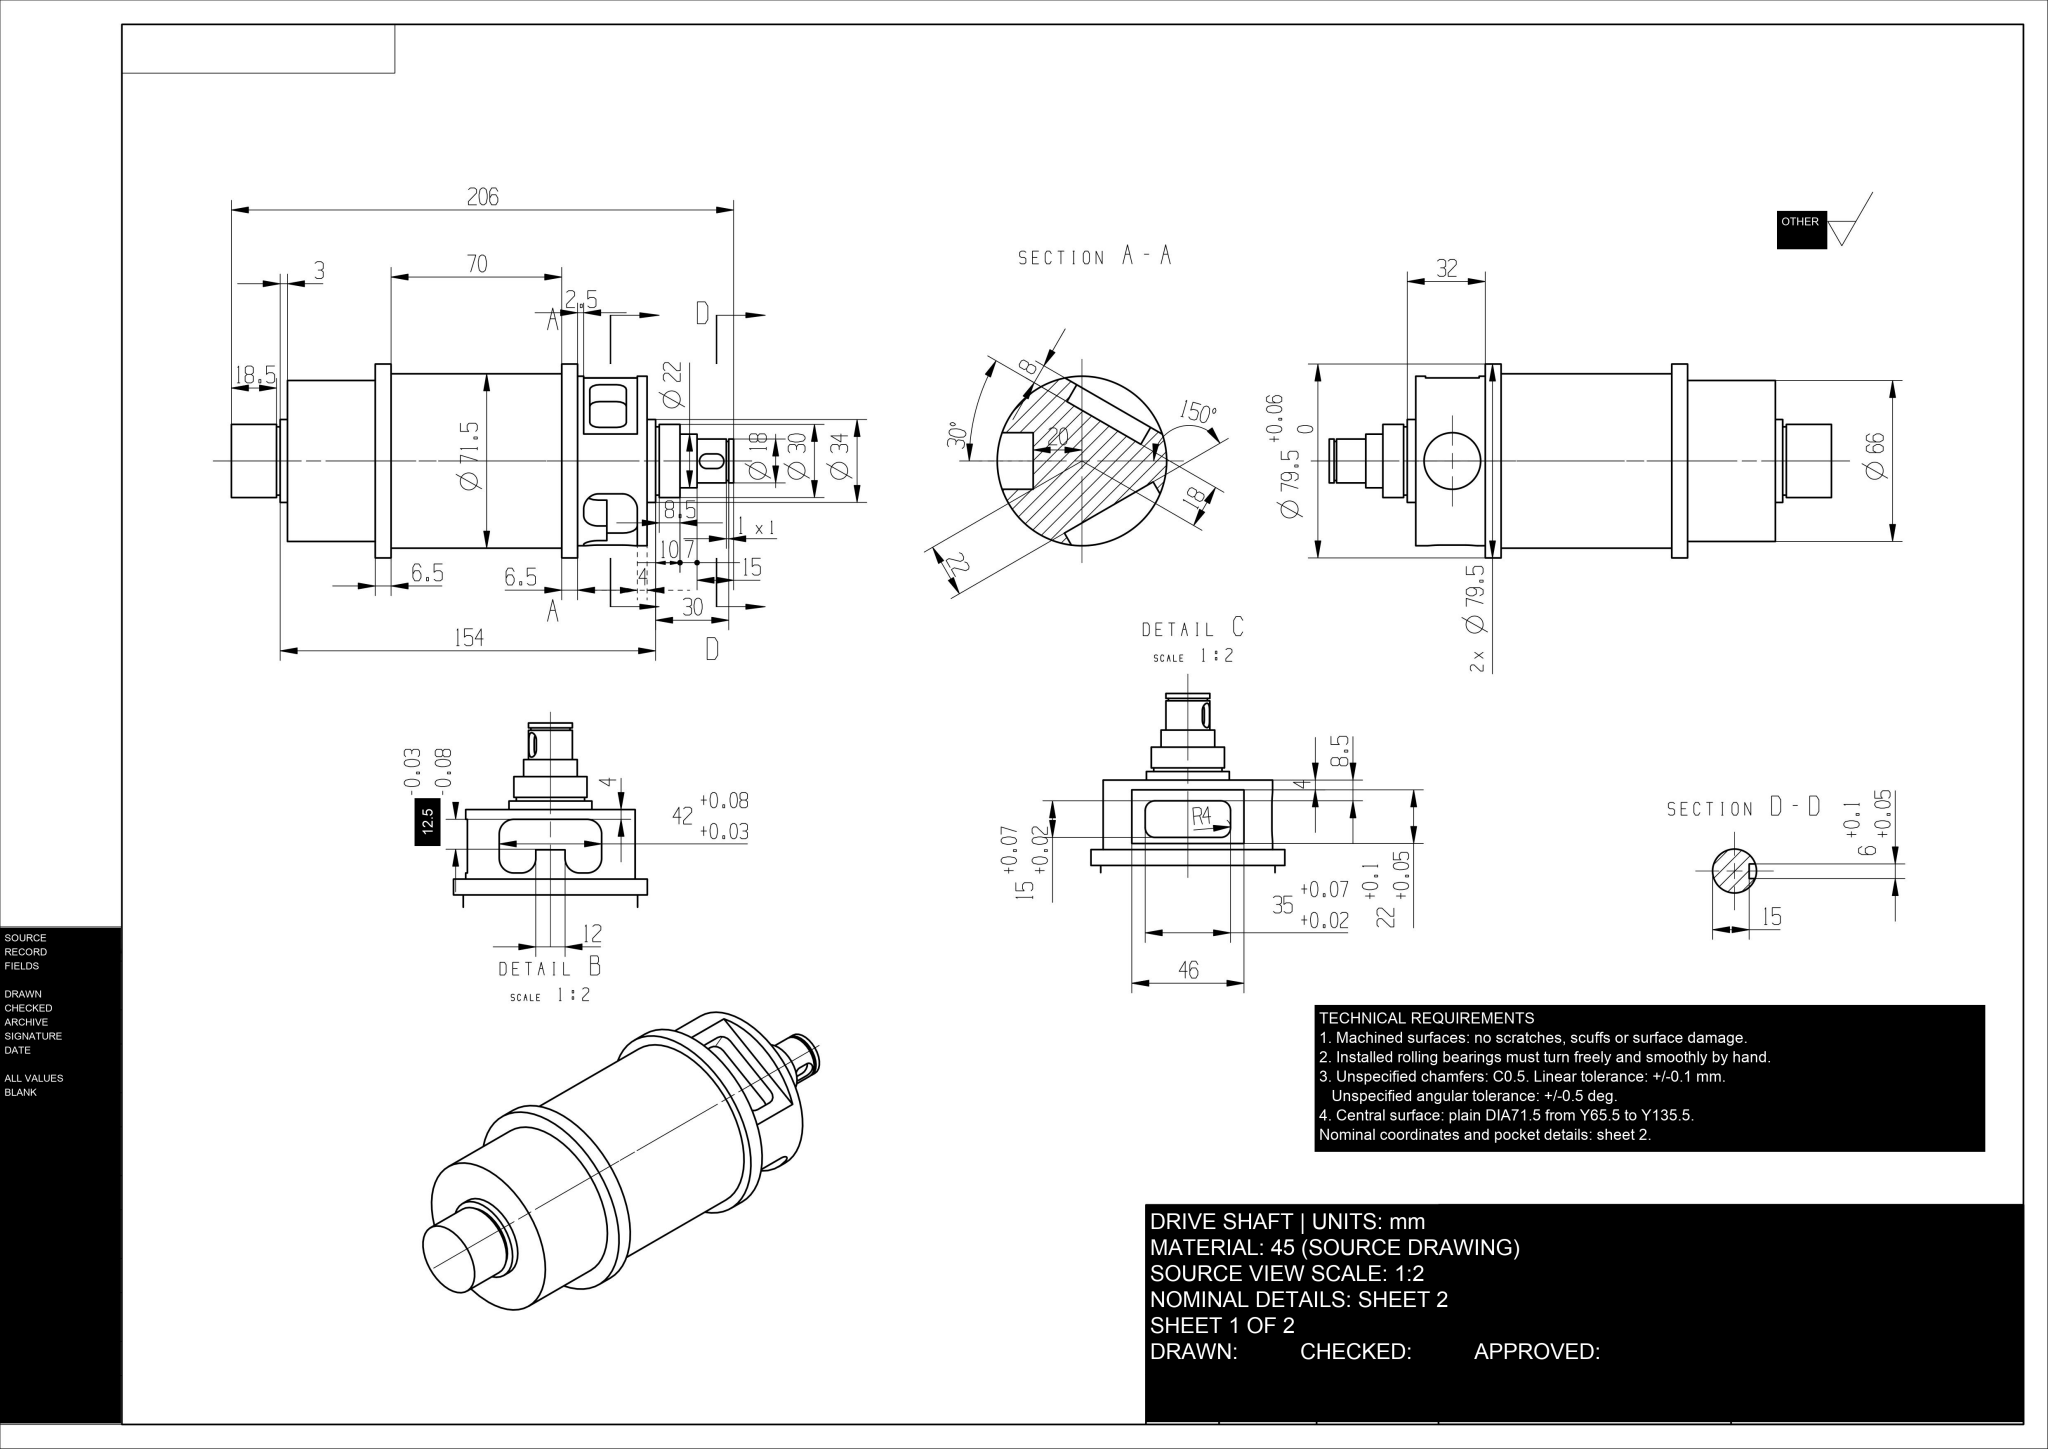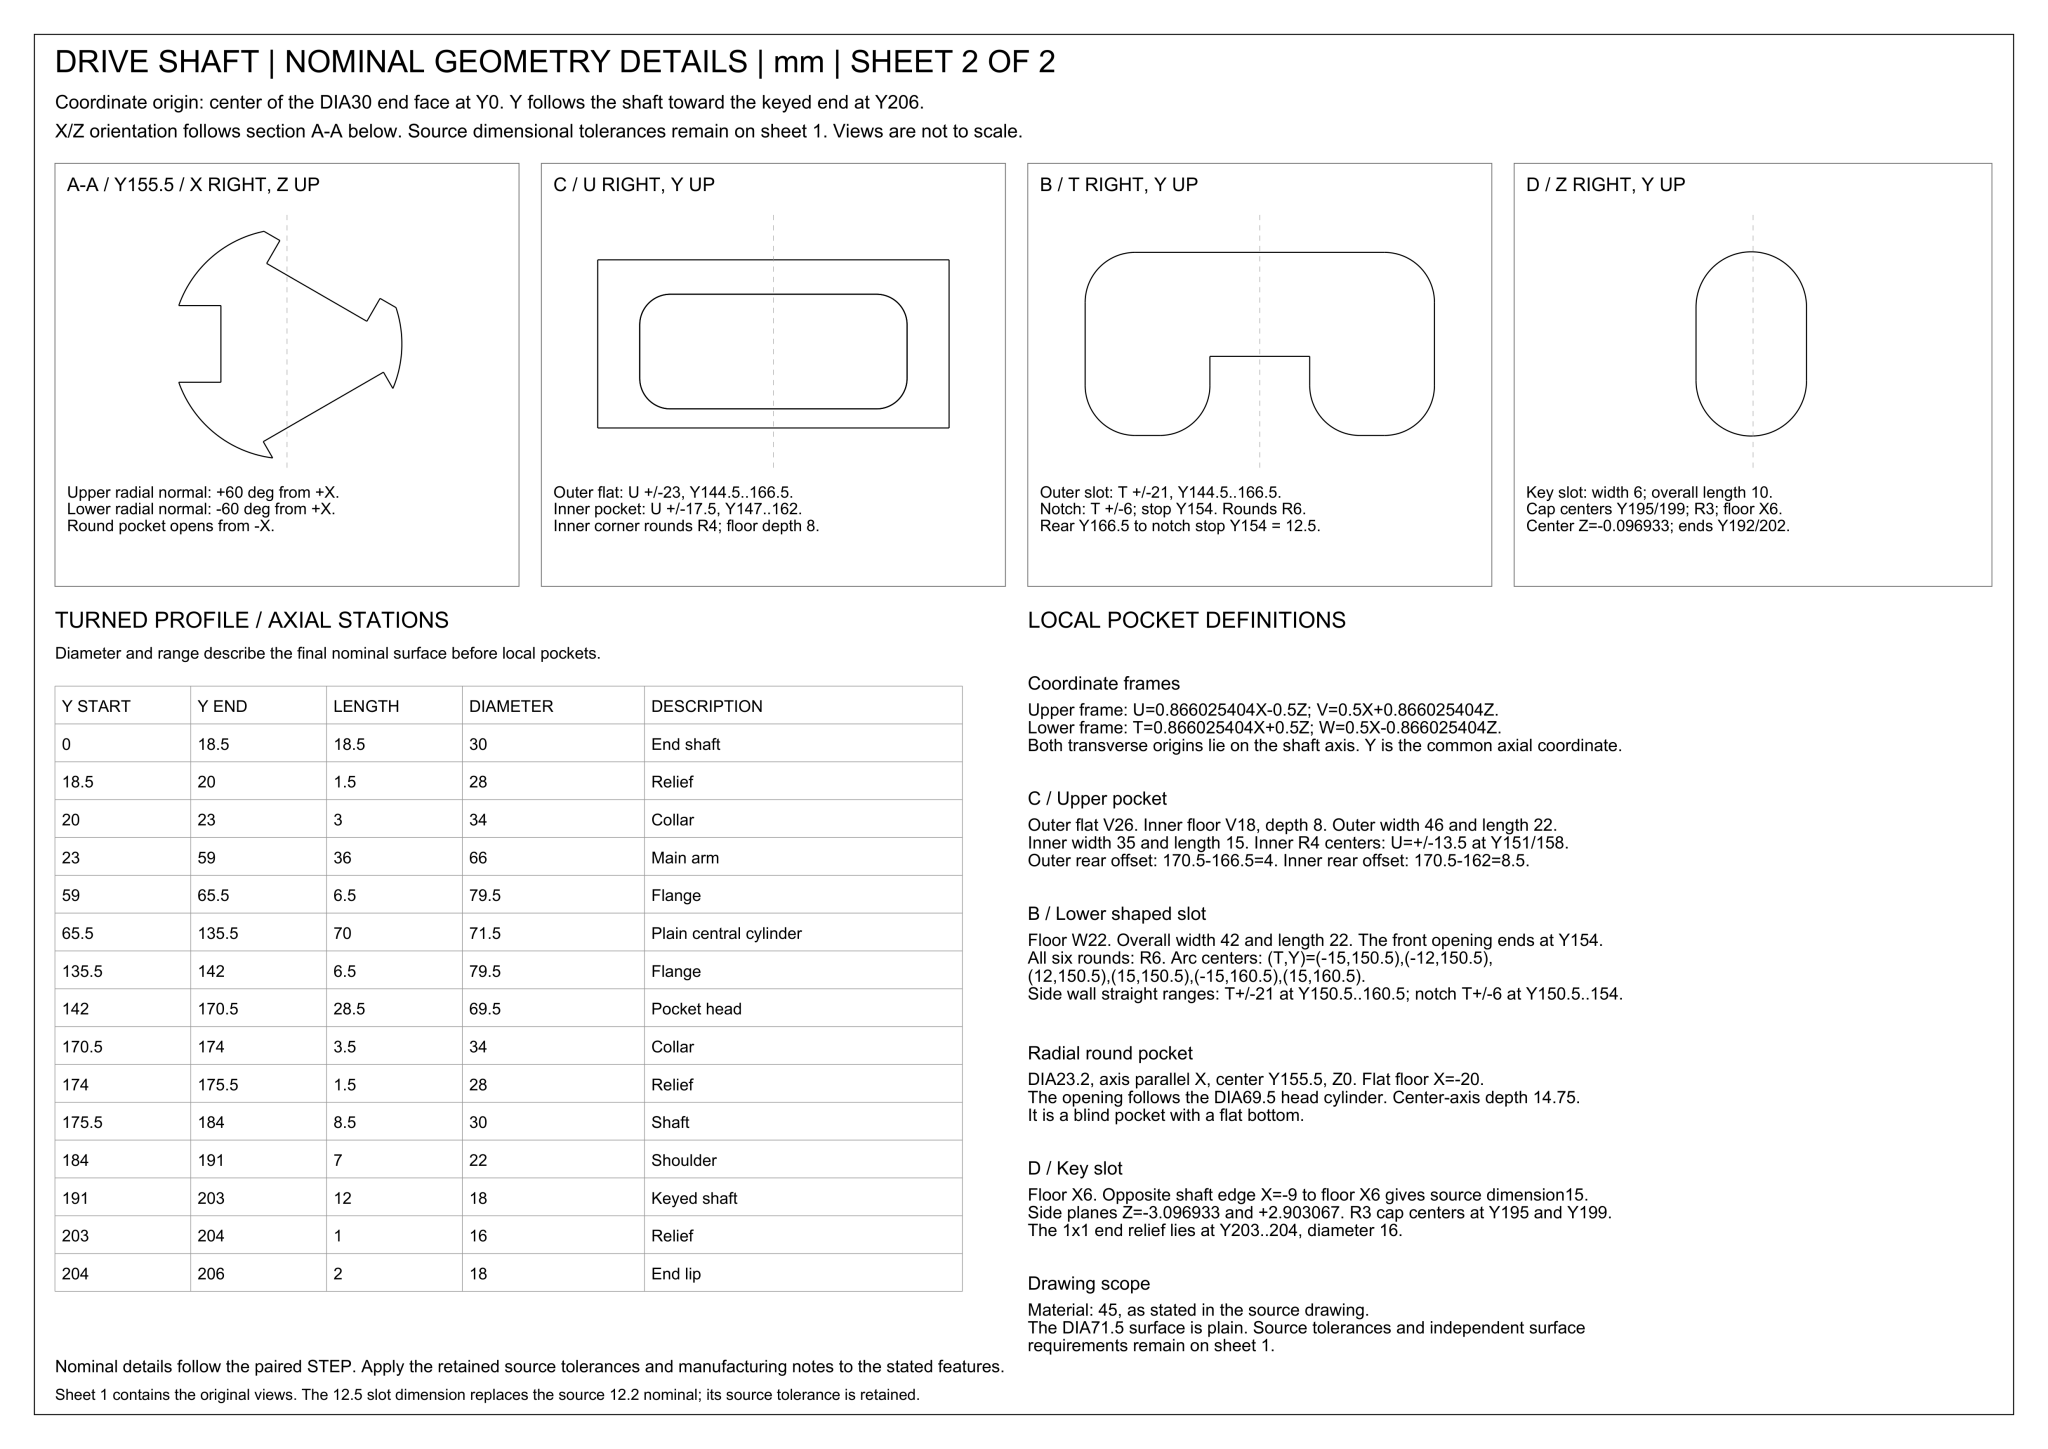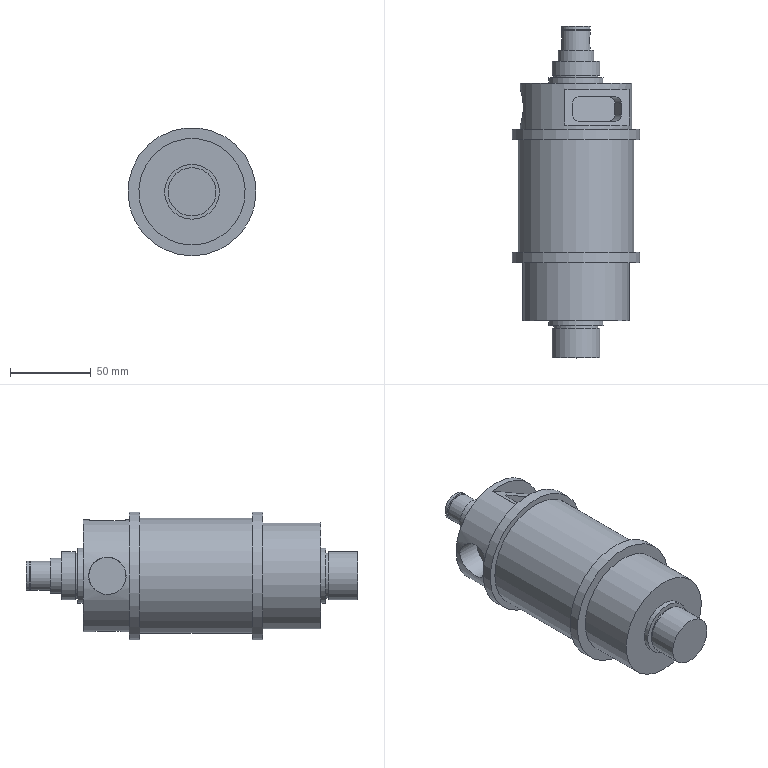Part | NX | mm | 1 solid | 67 faces | box 79.5 x 206 x 79.5 mm | volume 585909 mm3 | plane 39 | cylinder 28 | commonest cylinder face diameters 12 x6 8 x4 18 x2 79.5 x2 34 x2 28 x2 30 x2 6 x2